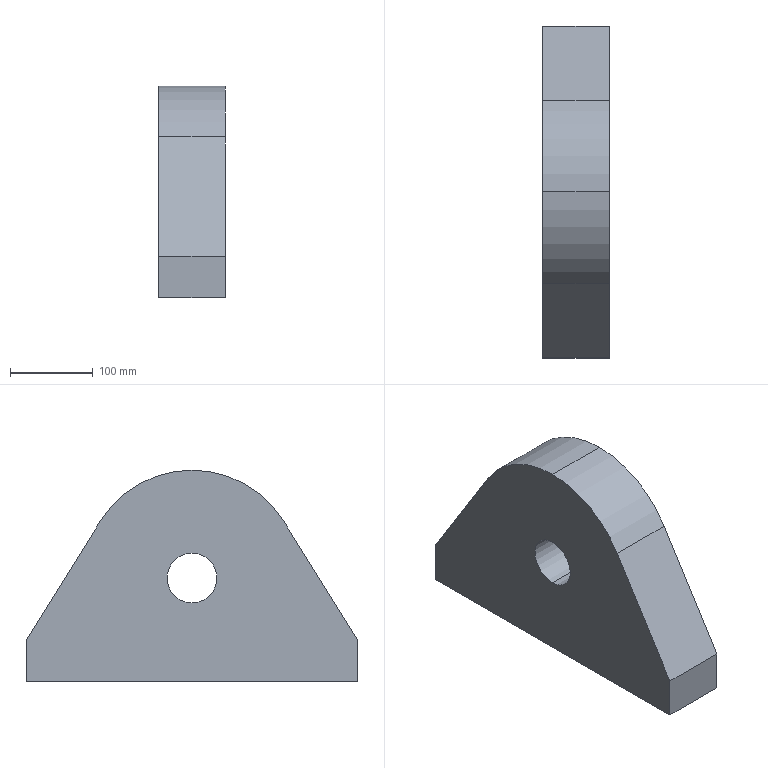Component | SolidWorks | Hanger-3_Hanger-1 | 1 solid | 11 faces | box 80 x 400 x 255 mm | volume 5706133 mm3 | plane 7 | cylinder 4 | commonest cylinder face diameters 60 x2 260 x2 | material Plain Carbon Steel
build123d program:
from build123d import *

# Parameters (mm, degrees)
SKETCH1_R           = 30
BOSS_EXTRUDE1_DEPTH = 40


with BuildPart() as part:
    # Sketch1 → Boss-Extrude1 (new, symmetric)
    with BuildSketch(Plane(origin=(0, 0, 0), x_dir=(1, 0, 0), z_dir=(0, 1, 0))):
        with BuildLine():
            Line((0, -75), (89.699, 68.802))
            ThreePointArc((89.699, 68.802), (200, 130), (310.301, 68.802))
            Line((310.301, 68.802), (400, -75))
            Line((400, -75), (400, -125))
            Line((400, -125), (0, -125))
            Line((0, -125), (0, -75))
        make_face()
        with Locations(Location((200, 0, 0), (0, 0, 270))):
            Circle(SKETCH1_R, mode=Mode.SUBTRACT)
    extrude(amount=BOSS_EXTRUDE1_DEPTH, both=True)


solid = part.part

# Placed as in the assembly
solid = solid.moved(Location((-5875.465, 3036.733, 6859.043), (180, 0, -90)))
STEP:
#1=COLOUR_RGB('',0.7922,0.8196,0.9333);
#2=FILL_AREA_STYLE_COLOUR('',#1);
#3=FILL_AREA_STYLE('',(#2));
#4=SURFACE_STYLE_FILL_AREA(#3);
#5=SURFACE_SIDE_STYLE('',(#4));
#6=SURFACE_STYLE_USAGE(.BOTH.,#5);
#7=PRESENTATION_STYLE_ASSIGNMENT((#6));
#8=CARTESIAN_POINT('',(-232.892,127.43,271.222));
#9=VERTEX_POINT('',#8);
#10=CARTESIAN_POINT('',(-232.892,127.43,268.86));
#11=VERTEX_POINT('',#10);
#12=CARTESIAN_POINT('',(-232.892,127.43,270.041));
#13=DIRECTION('',(-1.,-0.,-0.));
#14=DIRECTION('',(0.,0.,-1.));
#15=AXIS2_PLACEMENT_3D('',#12,#13,#14);
#16=CIRCLE('',#15,1.181);
#17=EDGE_CURVE('',#9,#11,#16,.T.);
#18=ORIENTED_EDGE('',*,*,#17,.T.);
#19=CARTESIAN_POINT('',(-229.743,127.43,268.86));
#20=VERTEX_POINT('',#19);
#21=CARTESIAN_POINT('',(-232.892,127.43,268.86));
#22=DIRECTION('',(1.,0.,0.));
#23=VECTOR('',#22,39.37);
#24=LINE('',#21,#23);
#25=EDGE_CURVE('',#11,#20,#24,.T.);
#26=ORIENTED_EDGE('',*,*,#25,.T.);
#27=CARTESIAN_POINT('',(-229.743,127.43,271.222));
#28=VERTEX_POINT('',#27);
#29=CARTESIAN_POINT('',(-229.743,127.43,270.041));
#30=DIRECTION('',(-1.,-0.,-0.));
#31=DIRECTION('',(0.,0.,-1.));
#32=AXIS2_PLACEMENT_3D('',#29,#30,#31);
#33=CIRCLE('',#32,1.181);
#34=EDGE_CURVE('',#28,#20,#33,.T.);
#35=ORIENTED_EDGE('',*,*,#34,.F.);
#36=CARTESIAN_POINT('',(-232.892,127.43,271.222));
#37=DIRECTION('',(1.,0.,0.));
#38=VECTOR('',#37,39.37);
#39=LINE('',#36,#38);
#40=EDGE_CURVE('',#9,#28,#39,.T.);
#41=ORIENTED_EDGE('',*,*,#40,.F.);
#42=EDGE_LOOP('',(#18,#26,#35,#41));
#43=FACE_OUTER_BOUND('',#42,.T.);
#44=CARTESIAN_POINT('',(-232.892,127.43,270.041));
#45=DIRECTION('',(1.,0.,0.));
#46=DIRECTION('',(0.,0.,1.));
#47=AXIS2_PLACEMENT_3D('',#44,#45,#46);
#48=CYLINDRICAL_SURFACE('',#47,1.181);
#49=ADVANCED_FACE('',(#43),#48,.F.);
#50=CARTESIAN_POINT('',(-232.892,127.43,275.159));
#51=VERTEX_POINT('',#50);
#52=CARTESIAN_POINT('',(-232.892,131.773,272.75));
#53=VERTEX_POINT('',#52);
#54=CARTESIAN_POINT('',(-232.892,127.43,270.041));
#55=DIRECTION('',(-1.,-0.,-0.));
#56=DIRECTION('',(0.,0.,-1.));
#57=AXIS2_PLACEMENT_3D('',#54,#55,#56);
#58=CIRCLE('',#57,5.118);
#59=EDGE_CURVE('',#51,#53,#58,.T.);
#60=ORIENTED_EDGE('',*,*,#59,.F.);
#61=CARTESIAN_POINT('',(-229.743,127.43,275.159));
#62=VERTEX_POINT('',#61);
#63=CARTESIAN_POINT('',(-232.892,127.43,275.159));
#64=DIRECTION('',(1.,0.,0.));
#65=VECTOR('',#64,39.37);
#66=LINE('',#63,#65);
#67=EDGE_CURVE('',#51,#62,#66,.T.);
#68=ORIENTED_EDGE('',*,*,#67,.T.);
#69=CARTESIAN_POINT('',(-229.743,131.773,272.75));
#70=VERTEX_POINT('',#69);
#71=CARTESIAN_POINT('',(-229.743,127.43,270.041));
#72=DIRECTION('',(-1.,-0.,-0.));
#73=DIRECTION('',(0.,0.,-1.));
#74=AXIS2_PLACEMENT_3D('',#71,#72,#73);
#75=CIRCLE('',#74,5.118);
#76=EDGE_CURVE('',#62,#70,#75,.T.);
#77=ORIENTED_EDGE('',*,*,#76,.T.);
#78=CARTESIAN_POINT('',(-232.892,131.773,272.75));
#79=DIRECTION('',(1.,0.,0.));
#80=VECTOR('',#79,39.37);
#81=LINE('',#78,#80);
#82=EDGE_CURVE('',#53,#70,#81,.T.);
#83=ORIENTED_EDGE('',*,*,#82,.F.);
#84=EDGE_LOOP('',(#60,#68,#77,#83));
#85=FACE_OUTER_BOUND('',#84,.T.);
#86=CARTESIAN_POINT('',(-232.892,127.43,270.041));
#87=DIRECTION('',(1.,0.,0.));
#88=DIRECTION('',(-0.,-0.,1.));
#89=AXIS2_PLACEMENT_3D('',#86,#87,#88);
#90=CYLINDRICAL_SURFACE('',#89,5.118);
#91=ADVANCED_FACE('',(#85),#90,.T.);
#92=CARTESIAN_POINT('',(-232.892,119.556,265.12));
#93=VERTEX_POINT('',#92);
#94=CARTESIAN_POINT('',(-232.892,119.556,267.088));
#95=VERTEX_POINT('',#94);
#96=CARTESIAN_POINT('',(-232.892,119.556,267.088));
#97=DIRECTION('',(-0.,-0.,1.));
#98=VECTOR('',#97,39.37);
#99=LINE('',#96,#98);
#100=EDGE_CURVE('',#93,#95,#99,.T.);
#101=ORIENTED_EDGE('',*,*,#100,.T.);
#102=CARTESIAN_POINT('',(-232.892,123.088,272.75));
#103=VERTEX_POINT('',#102);
#104=CARTESIAN_POINT('',(-232.892,119.556,267.088));
#105=DIRECTION('',(-0.,0.5292,0.8485));
#106=VECTOR('',#105,39.37);
#107=LINE('',#104,#106);
#108=EDGE_CURVE('',#95,#103,#107,.T.);
#109=ORIENTED_EDGE('',*,*,#108,.T.);
#110=CARTESIAN_POINT('',(-232.892,127.43,270.041));
#111=DIRECTION('',(-1.,-0.,-0.));
#112=DIRECTION('',(0.,0.,-1.));
#113=AXIS2_PLACEMENT_3D('',#110,#111,#112);
#114=CIRCLE('',#113,5.118);
#115=EDGE_CURVE('',#103,#51,#114,.T.);
#116=ORIENTED_EDGE('',*,*,#115,.T.);
#117=ORIENTED_EDGE('',*,*,#59,.T.);
#118=CARTESIAN_POINT('',(-232.892,135.304,267.088));
#119=VERTEX_POINT('',#118);
#120=CARTESIAN_POINT('',(-232.892,135.304,267.088));
#121=DIRECTION('',(0.,0.5292,-0.8485));
#122=VECTOR('',#121,39.37);
#123=LINE('',#120,#122);
#124=EDGE_CURVE('',#53,#119,#123,.T.);
#125=ORIENTED_EDGE('',*,*,#124,.T.);
#126=CARTESIAN_POINT('',(-232.892,135.304,265.12));
#127=VERTEX_POINT('',#126);
#128=CARTESIAN_POINT('',(-232.892,135.304,267.088));
#129=DIRECTION('',(0.,0.,-1.));
#130=VECTOR('',#129,39.37);
#131=LINE('',#128,#130);
#132=EDGE_CURVE('',#119,#127,#131,.T.);
#133=ORIENTED_EDGE('',*,*,#132,.T.);
#134=CARTESIAN_POINT('',(-232.892,135.304,265.12));
#135=DIRECTION('',(0.,-1.,-0.));
#136=VECTOR('',#135,39.37);
#137=LINE('',#134,#136);
#138=EDGE_CURVE('',#127,#93,#137,.T.);
#139=ORIENTED_EDGE('',*,*,#138,.T.);
#140=EDGE_LOOP('',(#101,#109,#116,#117,#125,#133,#139));
#141=FACE_OUTER_BOUND('',#140,.T.);
#142=ORIENTED_EDGE('',*,*,#17,.F.);
#143=CARTESIAN_POINT('',(-232.892,127.43,270.041));
#144=DIRECTION('',(-1.,-0.,-0.));
#145=DIRECTION('',(0.,0.,-1.));
#146=AXIS2_PLACEMENT_3D('',#143,#144,#145);
#147=CIRCLE('',#146,1.181);
#148=EDGE_CURVE('',#11,#9,#147,.T.);
#149=ORIENTED_EDGE('',*,*,#148,.F.);
#150=EDGE_LOOP('',(#142,#149));
#151=FACE_BOUND('',#150,.T.);
#152=CARTESIAN_POINT('',(-232.892,127.43,270.041));
#153=DIRECTION('',(-1.,-0.,-0.));
#154=DIRECTION('',(0.,0.,-1.));
#155=AXIS2_PLACEMENT_3D('',#152,#153,#154);
#156=PLANE('',#155);
#157=ADVANCED_FACE('',(#141,#151),#156,.T.);
#158=CARTESIAN_POINT('',(-229.743,119.556,265.12));
#159=VERTEX_POINT('',#158);
#160=CARTESIAN_POINT('',(-229.743,119.556,267.088));
#161=VERTEX_POINT('',#160);
#162=CARTESIAN_POINT('',(-229.743,119.556,267.088));
#163=DIRECTION('',(-0.,-0.,1.));
#164=VECTOR('',#163,39.37);
#165=LINE('',#162,#164);
#166=EDGE_CURVE('',#159,#161,#165,.T.);
#167=ORIENTED_EDGE('',*,*,#166,.F.);
#168=CARTESIAN_POINT('',(-229.743,135.304,265.12));
#169=VERTEX_POINT('',#168);
#170=CARTESIAN_POINT('',(-229.743,135.304,265.12));
#171=DIRECTION('',(0.,-1.,-0.));
#172=VECTOR('',#171,39.37);
#173=LINE('',#170,#172);
#174=EDGE_CURVE('',#169,#159,#173,.T.);
#175=ORIENTED_EDGE('',*,*,#174,.F.);
#176=CARTESIAN_POINT('',(-229.743,135.304,267.088));
#177=VERTEX_POINT('',#176);
#178=CARTESIAN_POINT('',(-229.743,135.304,267.088));
#179=DIRECTION('',(0.,0.,-1.));
#180=VECTOR('',#179,39.37);
#181=LINE('',#178,#180);
#182=EDGE_CURVE('',#177,#169,#181,.T.);
#183=ORIENTED_EDGE('',*,*,#182,.F.);
#184=CARTESIAN_POINT('',(-229.743,135.304,267.088));
#185=DIRECTION('',(0.,0.5292,-0.8485));
#186=VECTOR('',#185,39.37);
#187=LINE('',#184,#186);
#188=EDGE_CURVE('',#70,#177,#187,.T.);
#189=ORIENTED_EDGE('',*,*,#188,.F.);
#190=ORIENTED_EDGE('',*,*,#76,.F.);
#191=CARTESIAN_POINT('',(-229.743,123.088,272.75));
#192=VERTEX_POINT('',#191);
#193=CARTESIAN_POINT('',(-229.743,127.43,270.041));
#194=DIRECTION('',(-1.,-0.,-0.));
#195=DIRECTION('',(0.,0.,-1.));
#196=AXIS2_PLACEMENT_3D('',#193,#194,#195);
#197=CIRCLE('',#196,5.118);
#198=EDGE_CURVE('',#192,#62,#197,.T.);
#199=ORIENTED_EDGE('',*,*,#198,.F.);
#200=CARTESIAN_POINT('',(-229.743,119.556,267.088));
#201=DIRECTION('',(-0.,0.5292,0.8485));
#202=VECTOR('',#201,39.37);
#203=LINE('',#200,#202);
#204=EDGE_CURVE('',#161,#192,#203,.T.);
#205=ORIENTED_EDGE('',*,*,#204,.F.);
#206=EDGE_LOOP('',(#167,#175,#183,#189,#190,#199,#205));
#207=FACE_OUTER_BOUND('',#206,.T.);
#208=ORIENTED_EDGE('',*,*,#34,.T.);
#209=CARTESIAN_POINT('',(-229.743,127.43,270.041));
#210=DIRECTION('',(-1.,-0.,-0.));
#211=DIRECTION('',(0.,0.,-1.));
#212=AXIS2_PLACEMENT_3D('',#209,#210,#211);
#213=CIRCLE('',#212,1.181);
#214=EDGE_CURVE('',#20,#28,#213,.T.);
#215=ORIENTED_EDGE('',*,*,#214,.T.);
#216=EDGE_LOOP('',(#208,#215));
#217=FACE_BOUND('',#216,.T.);
#218=CARTESIAN_POINT('',(-229.743,127.43,270.041));
#219=DIRECTION('',(-1.,-0.,-0.));
#220=DIRECTION('',(0.,0.,-1.));
#221=AXIS2_PLACEMENT_3D('',#218,#219,#220);
#222=PLANE('',#221);
#223=ADVANCED_FACE('',(#207,#217),#222,.F.);
#224=ORIENTED_EDGE('',*,*,#166,.T.);
#225=CARTESIAN_POINT('',(-232.892,119.556,267.088));
#226=DIRECTION('',(1.,0.,0.));
#227=VECTOR('',#226,39.37);
#228=LINE('',#225,#227);
#229=EDGE_CURVE('',#95,#161,#228,.T.);
#230=ORIENTED_EDGE('',*,*,#229,.F.);
#231=ORIENTED_EDGE('',*,*,#100,.F.);
#232=CARTESIAN_POINT('',(-232.892,119.556,265.12));
#233=DIRECTION('',(1.,0.,0.));
#234=VECTOR('',#233,39.37);
#235=LINE('',#232,#234);
#236=EDGE_CURVE('',#93,#159,#235,.T.);
#237=ORIENTED_EDGE('',*,*,#236,.T.);
#238=EDGE_LOOP('',(#224,#230,#231,#237));
#239=FACE_OUTER_BOUND('',#238,.T.);
#240=CARTESIAN_POINT('',(-232.892,119.556,267.088));
#241=DIRECTION('',(-0.,1.,0.));
#242=DIRECTION('',(0.,0.,-1.));
#243=AXIS2_PLACEMENT_3D('',#240,#241,#242);
#244=PLANE('',#243);
#245=ADVANCED_FACE('',(#239),#244,.F.);
#246=ORIENTED_EDGE('',*,*,#204,.T.);
#247=CARTESIAN_POINT('',(-232.892,123.088,272.75));
#248=DIRECTION('',(1.,0.,0.));
#249=VECTOR('',#248,39.37);
#250=LINE('',#247,#249);
#251=EDGE_CURVE('',#103,#192,#250,.T.);
#252=ORIENTED_EDGE('',*,*,#251,.F.);
#253=ORIENTED_EDGE('',*,*,#108,.F.);
#254=ORIENTED_EDGE('',*,*,#229,.T.);
#255=EDGE_LOOP('',(#246,#252,#253,#254));
#256=FACE_OUTER_BOUND('',#255,.T.);
#257=CARTESIAN_POINT('',(-232.892,119.556,267.088));
#258=DIRECTION('',(0.,0.8485,-0.5292));
#259=DIRECTION('',(0.,-0.5292,-0.8485));
#260=AXIS2_PLACEMENT_3D('',#257,#258,#259);
#261=PLANE('',#260);
#262=ADVANCED_FACE('',(#256),#261,.F.);
#263=ORIENTED_EDGE('',*,*,#67,.F.);
#264=ORIENTED_EDGE('',*,*,#115,.F.);
#265=ORIENTED_EDGE('',*,*,#251,.T.);
#266=ORIENTED_EDGE('',*,*,#198,.T.);
#267=EDGE_LOOP('',(#263,#264,#265,#266));
#268=FACE_OUTER_BOUND('',#267,.T.);
#269=CARTESIAN_POINT('',(-232.892,127.43,270.041));
#270=DIRECTION('',(1.,0.,0.));
#271=DIRECTION('',(-0.,-0.,1.));
#272=AXIS2_PLACEMENT_3D('',#269,#270,#271);
#273=CYLINDRICAL_SURFACE('',#272,5.118);
#274=ADVANCED_FACE('',(#268),#273,.T.);
#275=ORIENTED_EDGE('',*,*,#188,.T.);
#276=CARTESIAN_POINT('',(-232.892,135.304,267.088));
#277=DIRECTION('',(1.,0.,0.));
#278=VECTOR('',#277,39.37);
#279=LINE('',#276,#278);
#280=EDGE_CURVE('',#119,#177,#279,.T.);
#281=ORIENTED_EDGE('',*,*,#280,.F.);
#282=ORIENTED_EDGE('',*,*,#124,.F.);
#283=ORIENTED_EDGE('',*,*,#82,.T.);
#284=EDGE_LOOP('',(#275,#281,#282,#283));
#285=FACE_OUTER_BOUND('',#284,.T.);
#286=CARTESIAN_POINT('',(-232.892,135.304,267.088));
#287=DIRECTION('',(0.,-0.8485,-0.5292));
#288=DIRECTION('',(-0.,-0.5292,0.8485));
#289=AXIS2_PLACEMENT_3D('',#286,#287,#288);
#290=PLANE('',#289);
#291=ADVANCED_FACE('',(#285),#290,.F.);
#292=ORIENTED_EDGE('',*,*,#182,.T.);
#293=CARTESIAN_POINT('',(-232.892,135.304,265.12));
#294=DIRECTION('',(1.,0.,0.));
#295=VECTOR('',#294,39.37);
#296=LINE('',#293,#295);
#297=EDGE_CURVE('',#127,#169,#296,.T.);
#298=ORIENTED_EDGE('',*,*,#297,.F.);
#299=ORIENTED_EDGE('',*,*,#132,.F.);
#300=ORIENTED_EDGE('',*,*,#280,.T.);
#301=EDGE_LOOP('',(#292,#298,#299,#300));
#302=FACE_OUTER_BOUND('',#301,.T.);
#303=CARTESIAN_POINT('',(-232.892,135.304,267.088));
#304=DIRECTION('',(0.,-1.,-0.));
#305=DIRECTION('',(-0.,-0.,1.));
#306=AXIS2_PLACEMENT_3D('',#303,#304,#305);
#307=PLANE('',#306);
#308=ADVANCED_FACE('',(#302),#307,.F.);
#309=ORIENTED_EDGE('',*,*,#174,.T.);
#310=ORIENTED_EDGE('',*,*,#236,.F.);
#311=ORIENTED_EDGE('',*,*,#138,.F.);
#312=ORIENTED_EDGE('',*,*,#297,.T.);
#313=EDGE_LOOP('',(#309,#310,#311,#312));
#314=FACE_OUTER_BOUND('',#313,.T.);
#315=CARTESIAN_POINT('',(-232.892,135.304,265.12));
#316=DIRECTION('',(-0.,-0.,1.));
#317=DIRECTION('',(-0.,1.,0.));
#318=AXIS2_PLACEMENT_3D('',#315,#316,#317);
#319=PLANE('',#318);
#320=ADVANCED_FACE('',(#314),#319,.F.);
#321=ORIENTED_EDGE('',*,*,#25,.F.);
#322=ORIENTED_EDGE('',*,*,#148,.T.);
#323=ORIENTED_EDGE('',*,*,#40,.T.);
#324=ORIENTED_EDGE('',*,*,#214,.F.);
#325=EDGE_LOOP('',(#321,#322,#323,#324));
#326=FACE_OUTER_BOUND('',#325,.T.);
#327=CARTESIAN_POINT('',(-232.892,127.43,270.041));
#328=DIRECTION('',(1.,0.,0.));
#329=DIRECTION('',(0.,0.,1.));
#330=AXIS2_PLACEMENT_3D('',#327,#328,#329);
#331=CYLINDRICAL_SURFACE('',#330,1.181);
#332=ADVANCED_FACE('',(#326),#331,.F.);
#333=CLOSED_SHELL('',(#49,#91,#157,#223,#245,#262,#274,#291,#308,#320,#332));
#334=MANIFOLD_SOLID_BREP('',#333);
#335=STYLED_ITEM('',(#7),#334);
#336=(LENGTH_UNIT()NAMED_UNIT(*)SI_UNIT($,.METRE.));
#337=LENGTH_MEASURE_WITH_UNIT(LENGTH_MEASURE(0.0254),#336);
#338=DIMENSIONAL_EXPONENTS(1.,0.,0.,0.,0.,0.,0.);
#339=(CONVERSION_BASED_UNIT('',#337)LENGTH_UNIT()NAMED_UNIT(#338));
#340=UNCERTAINTY_MEASURE_WITH_UNIT(LENGTH_MEASURE(0.00001),#339,'','');
#341=(NAMED_UNIT(*)PLANE_ANGLE_UNIT()SI_UNIT($,.RADIAN.));
#342=(NAMED_UNIT(*)SI_UNIT($,.STERADIAN.)SOLID_ANGLE_UNIT());
#343=(GEOMETRIC_REPRESENTATION_CONTEXT(3)GLOBAL_UNCERTAINTY_ASSIGNED_CONTEXT((#340))GLOBAL_UNIT_ASSIGNED_CONTEXT((#339,#341,#342))REPRESENTATION_CONTEXT('',''));
#344=MECHANICAL_DESIGN_GEOMETRIC_PRESENTATION_REPRESENTATION('',(#335),#343);
#345=PRESENTATION_LAYER_ASSIGNMENT('','',(#335));
#346=CARTESIAN_POINT('',(0.,0.,0.));
#347=DIRECTION('',(0.,0.,1.));
#348=DIRECTION('',(1.,0.,0.));
#349=AXIS2_PLACEMENT_3D('',#346,#347,#348);
#350=(LENGTH_UNIT()NAMED_UNIT(*)SI_UNIT($,.METRE.));
#351=LENGTH_MEASURE_WITH_UNIT(LENGTH_MEASURE(0.0254),#350);
#352=DIMENSIONAL_EXPONENTS(1.,0.,0.,0.,0.,0.,0.);
#353=(CONVERSION_BASED_UNIT('',#351)LENGTH_UNIT()NAMED_UNIT(#352));
#354=UNCERTAINTY_MEASURE_WITH_UNIT(LENGTH_MEASURE(0.00001),#353,'','');
#355=(NAMED_UNIT(*)PLANE_ANGLE_UNIT()SI_UNIT($,.RADIAN.));
#356=(NAMED_UNIT(*)SI_UNIT($,.STERADIAN.)SOLID_ANGLE_UNIT());
#357=(GEOMETRIC_REPRESENTATION_CONTEXT(3)GLOBAL_UNCERTAINTY_ASSIGNED_CONTEXT((#354))GLOBAL_UNIT_ASSIGNED_CONTEXT((#353,#355,#356))REPRESENTATION_CONTEXT('',''));
#358=ADVANCED_BREP_SHAPE_REPRESENTATION('',(#334,#349),#357);